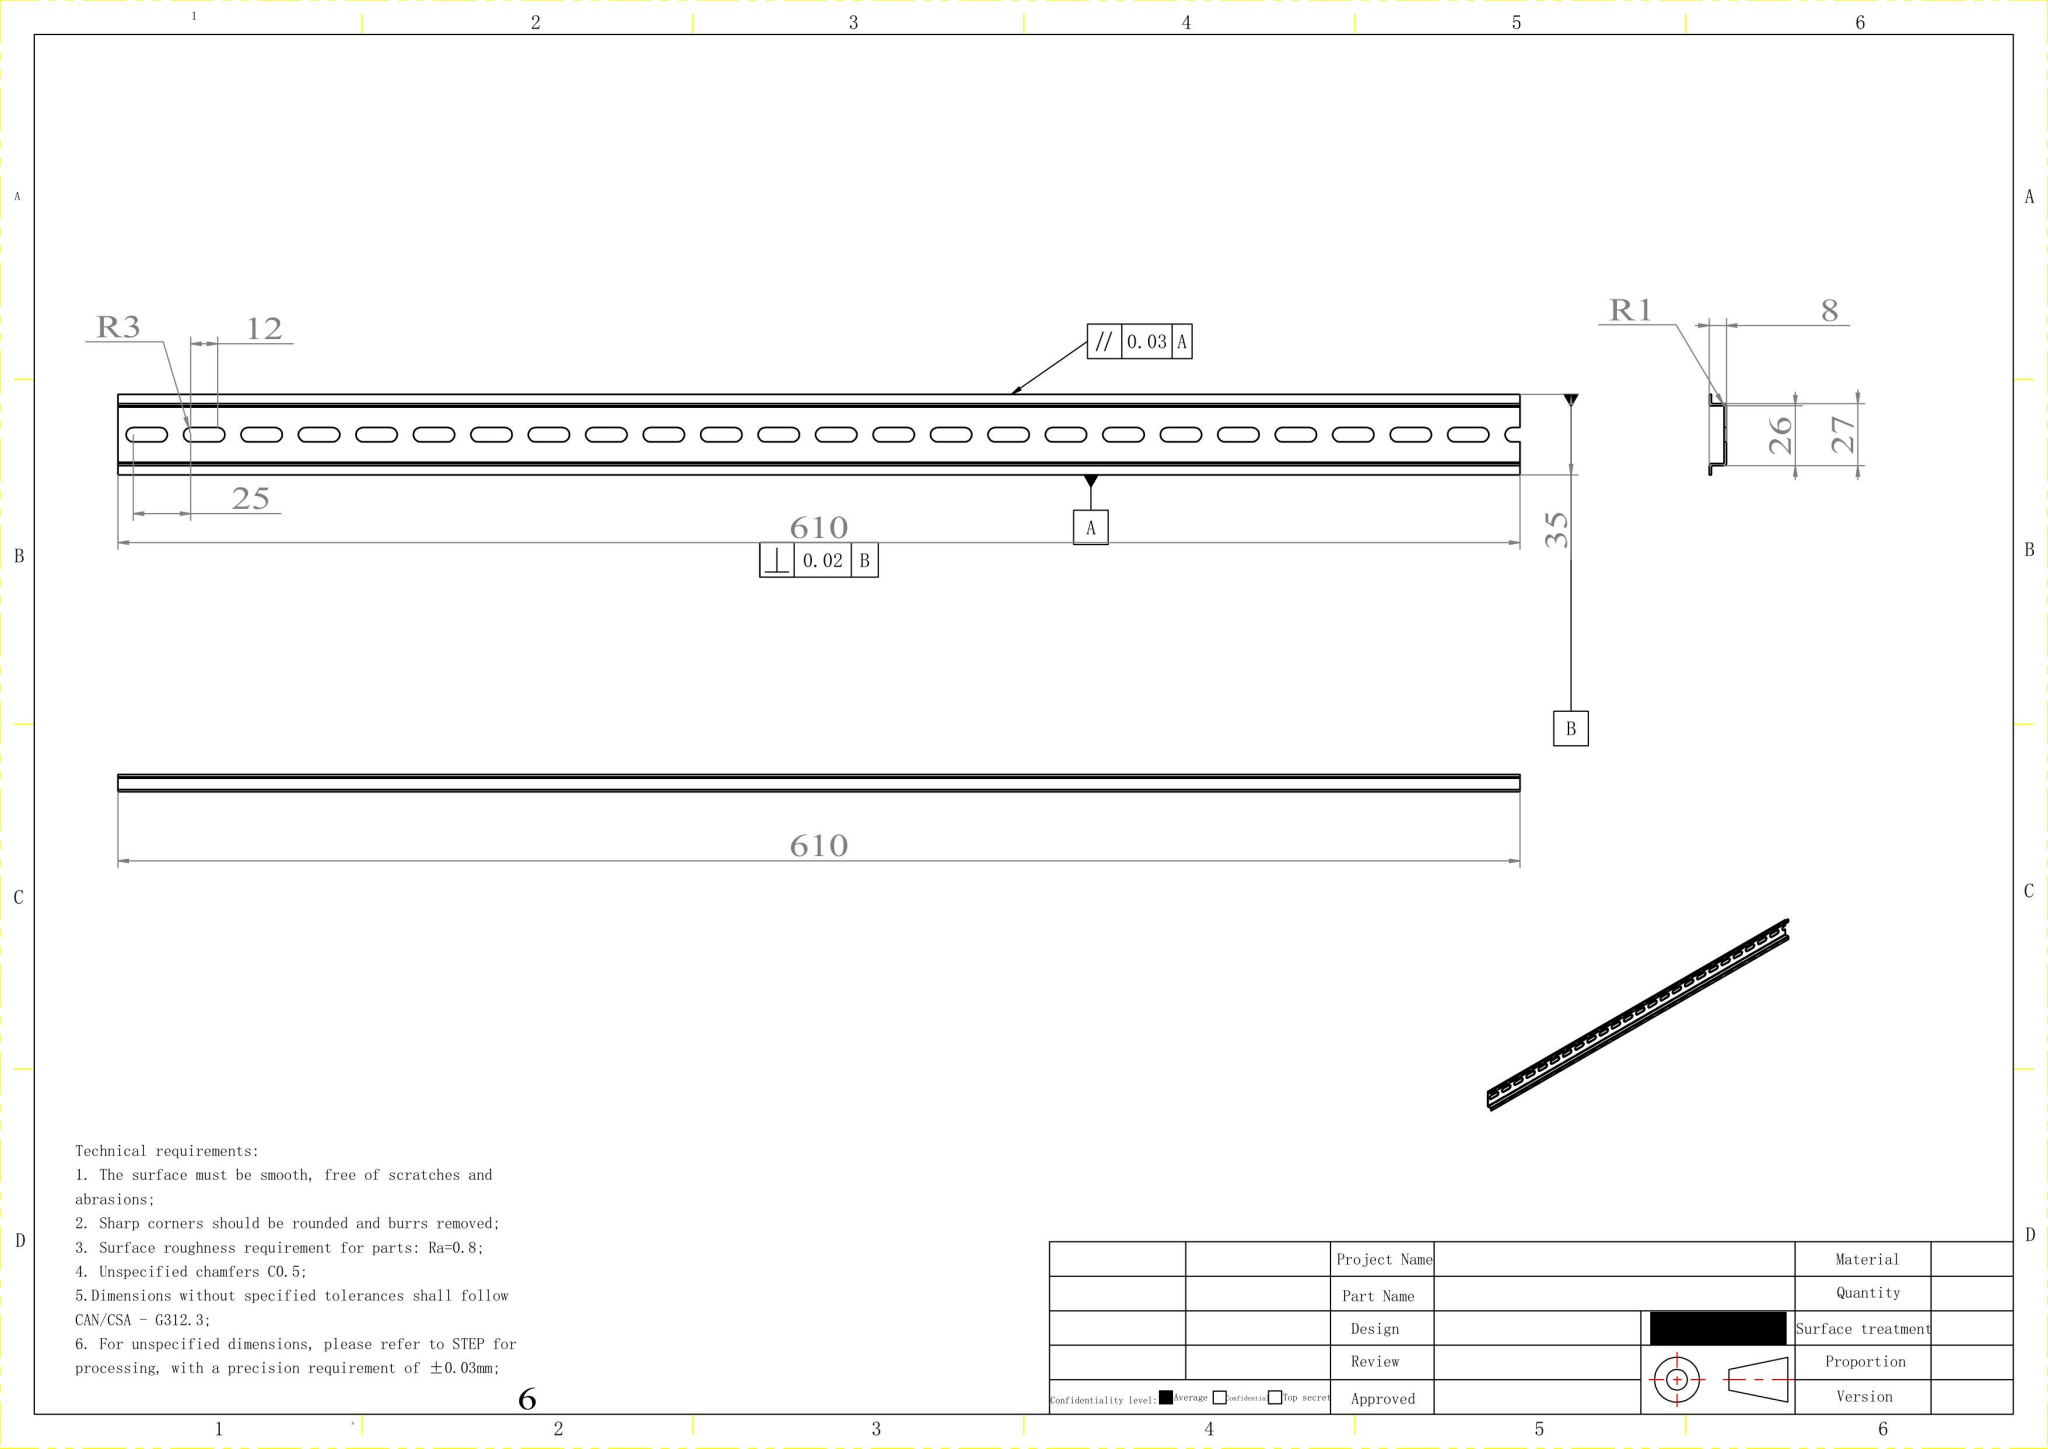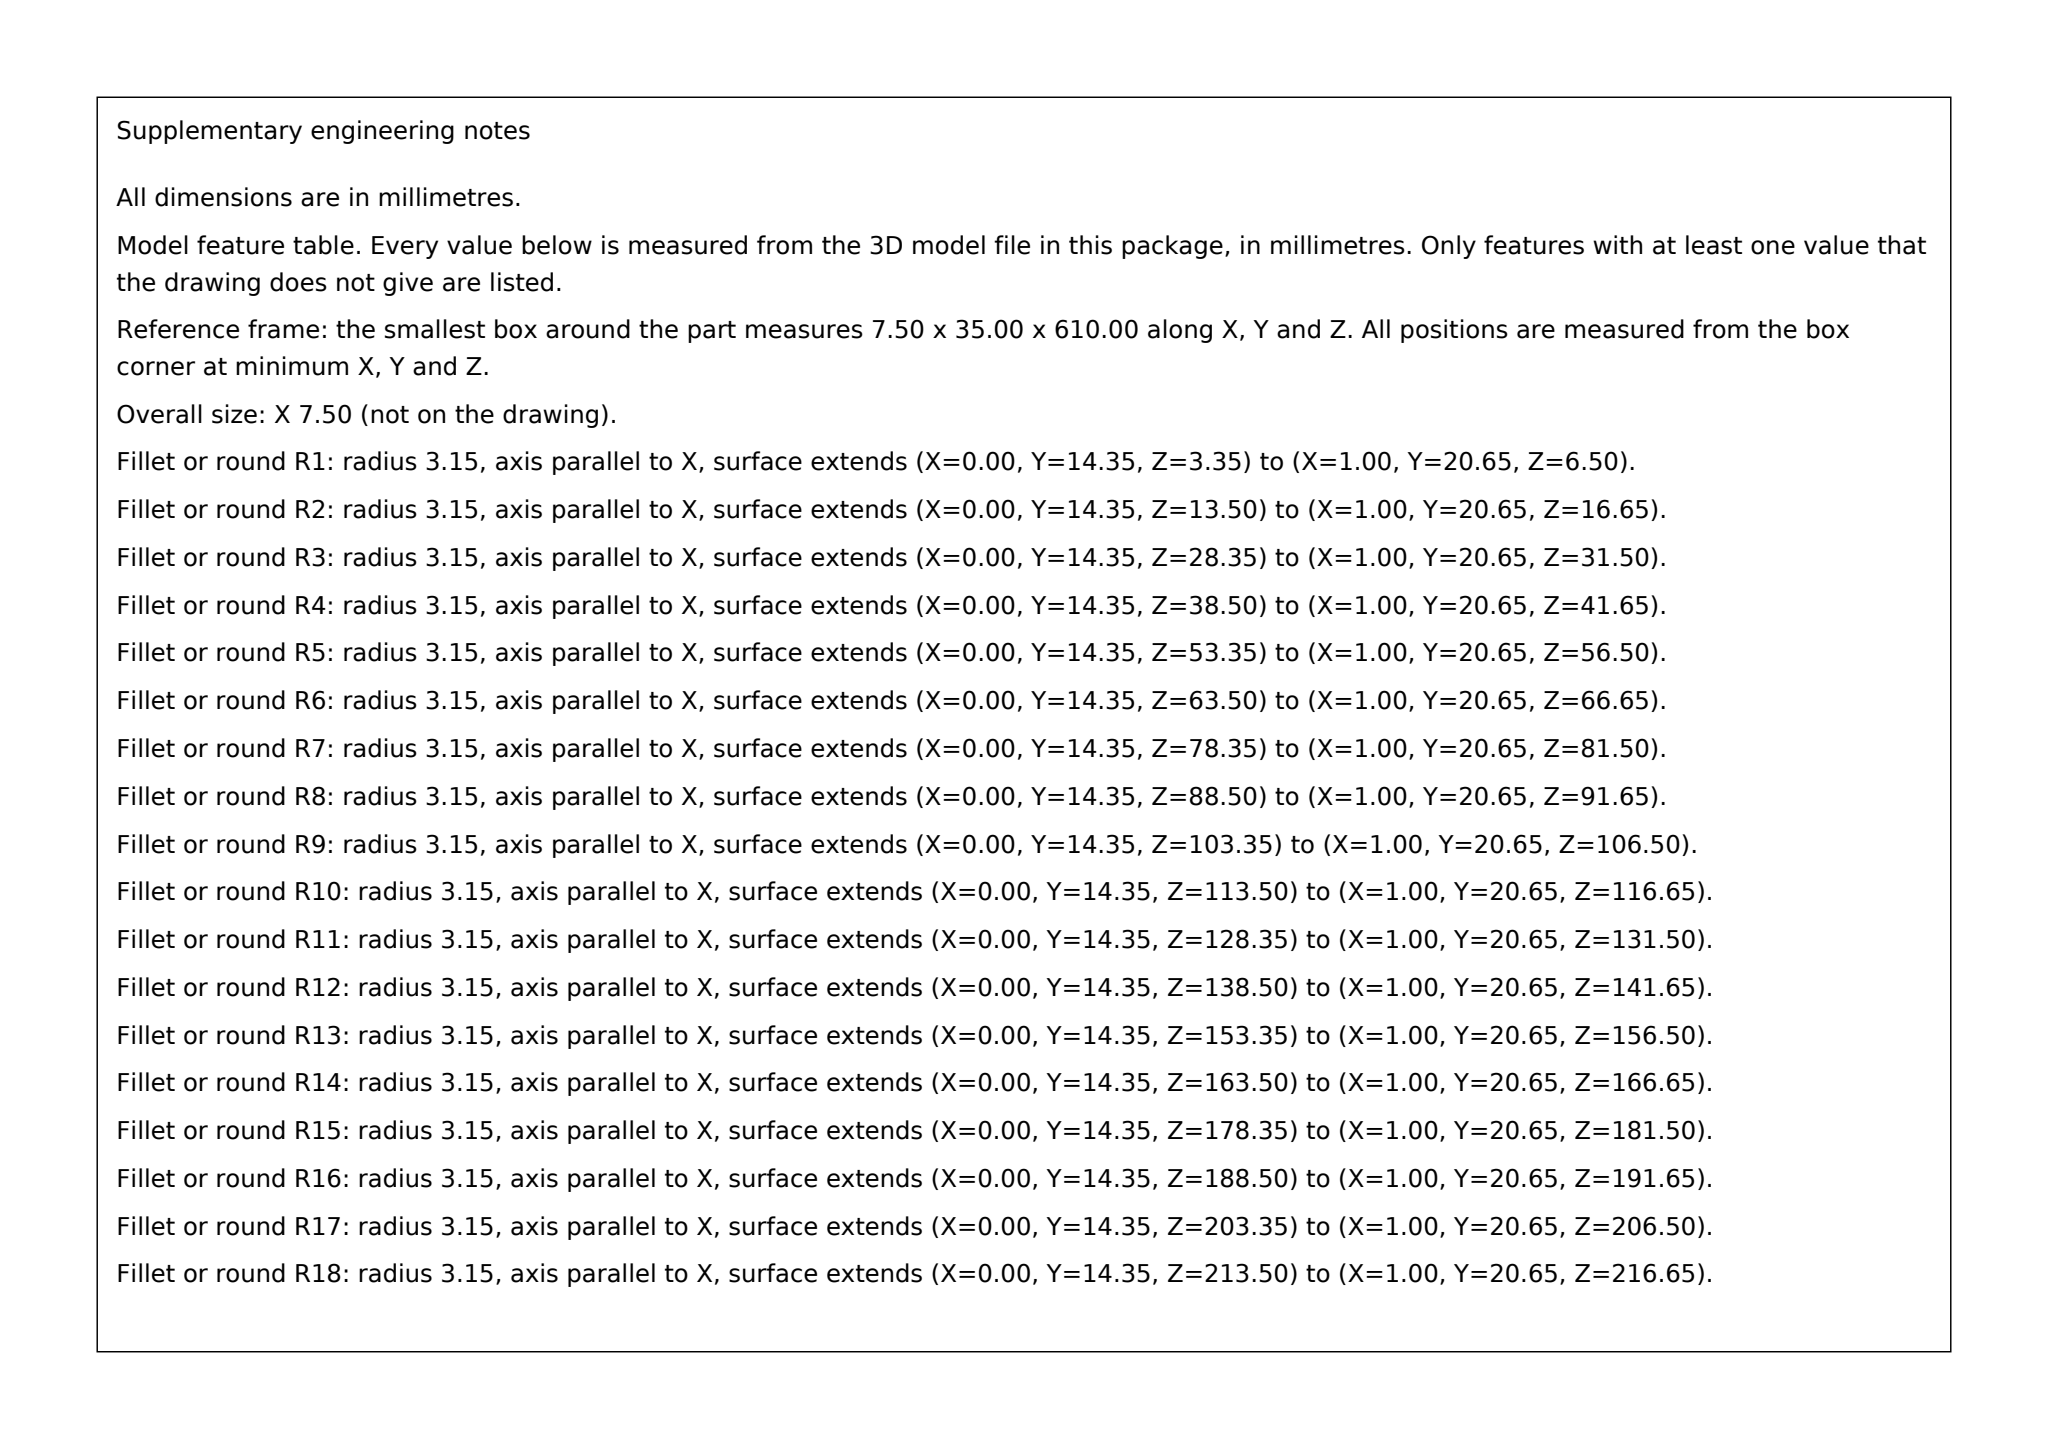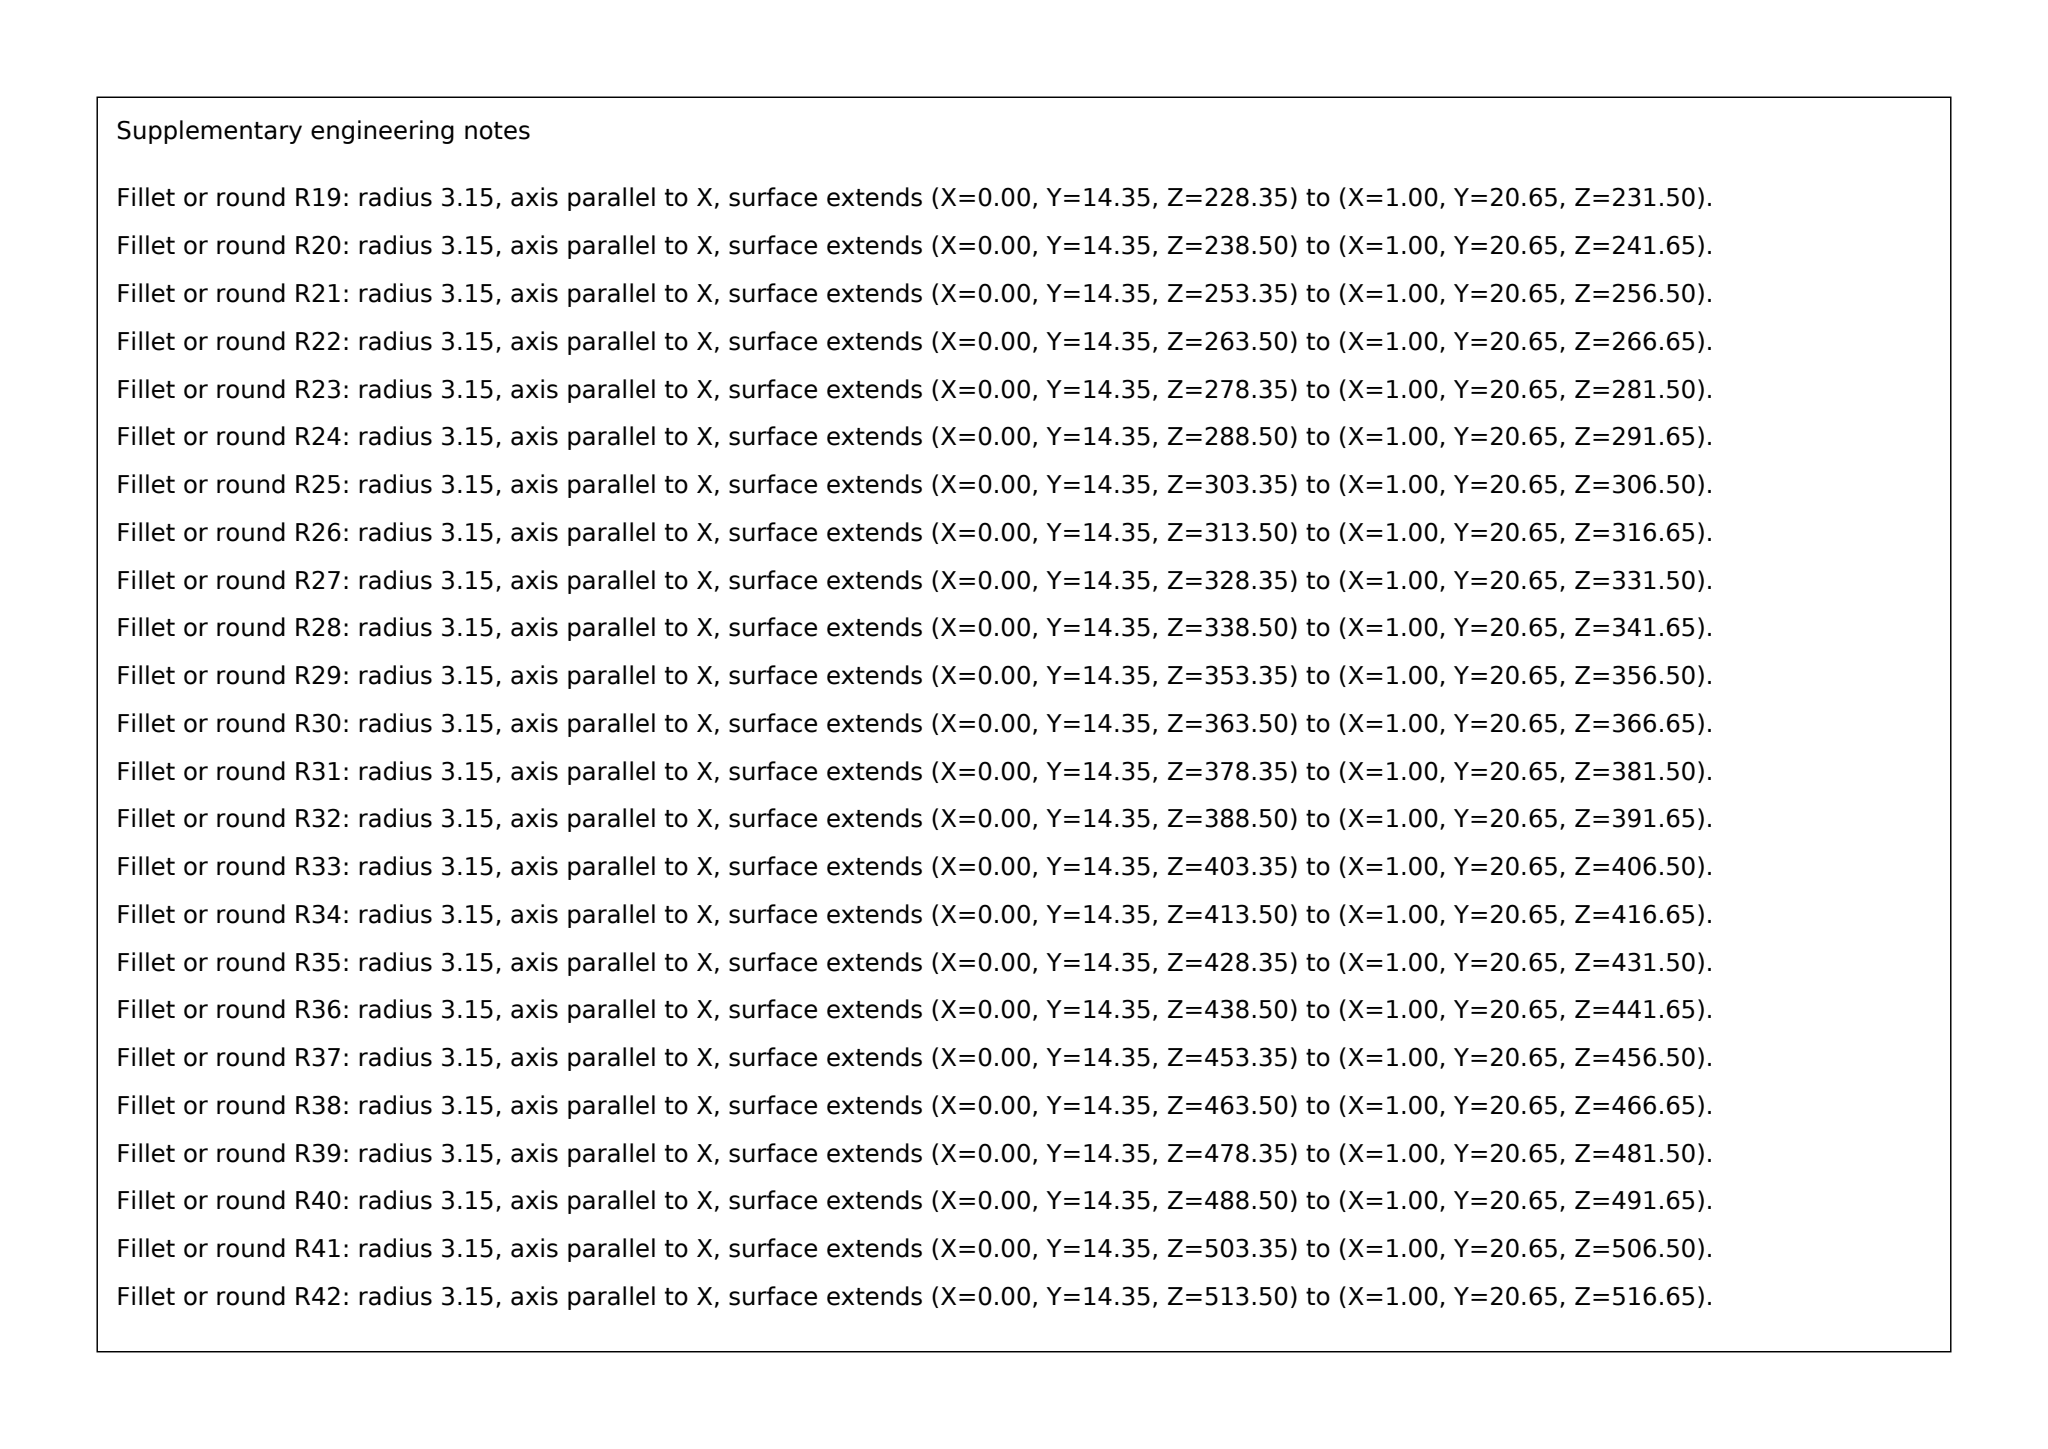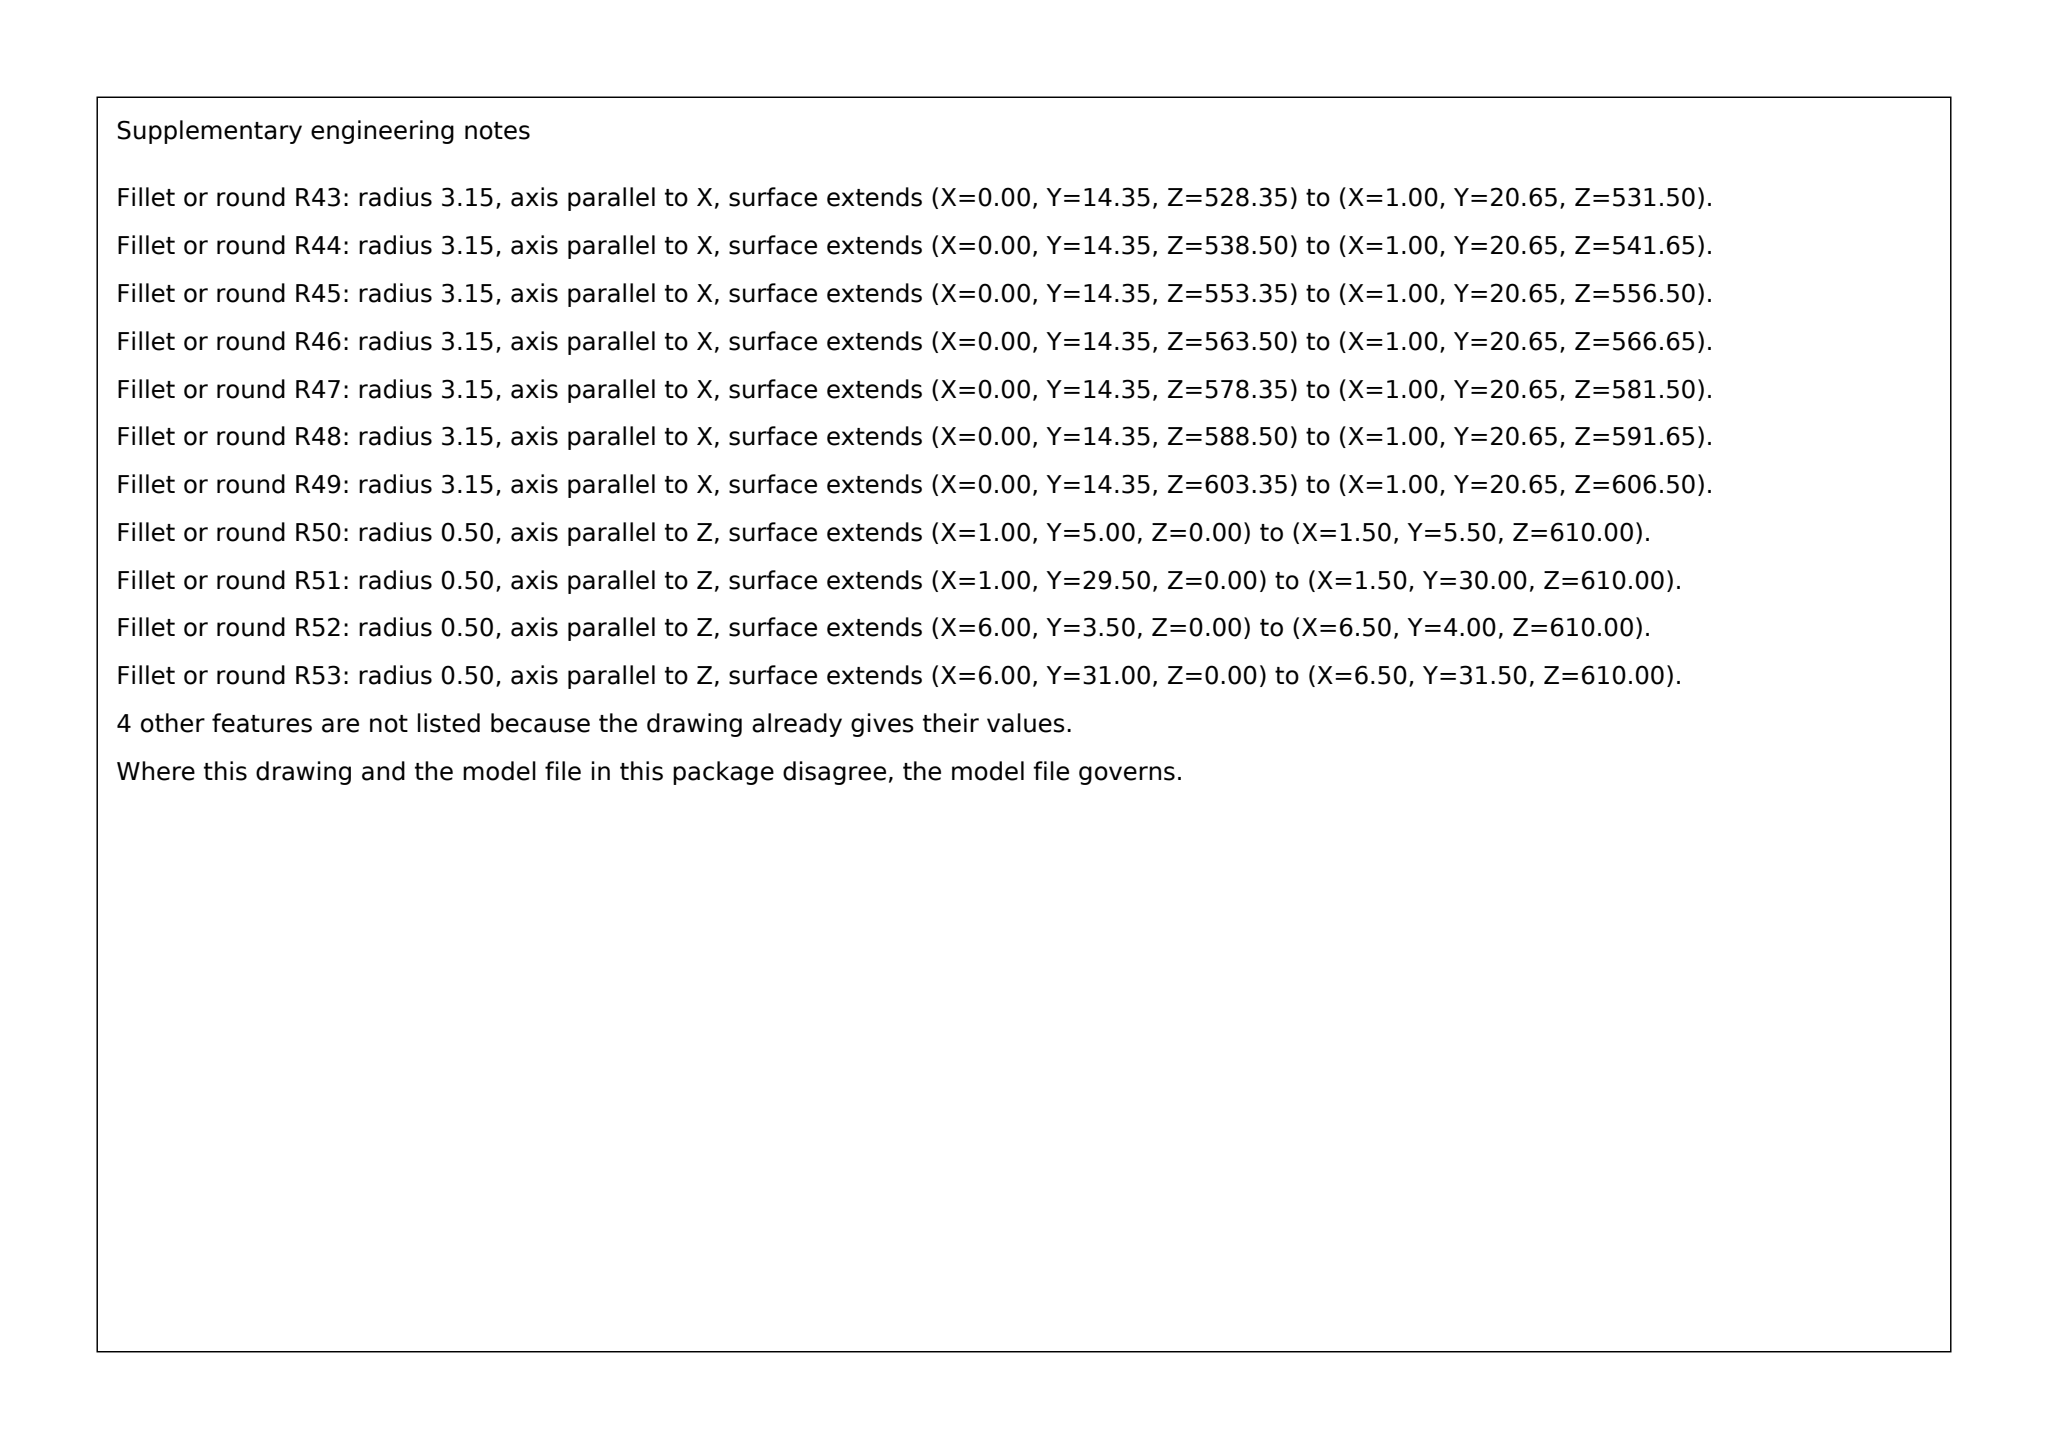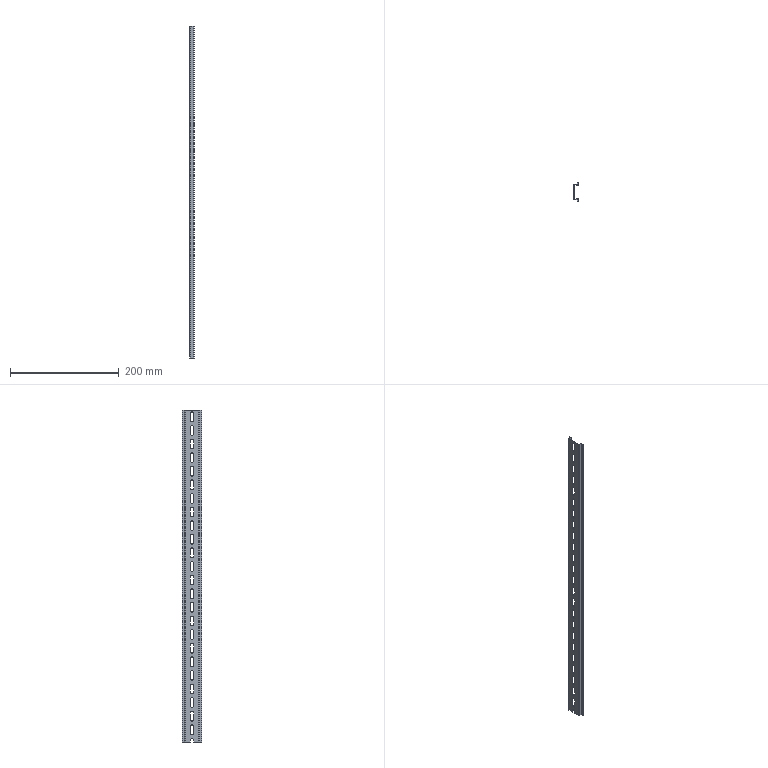Part | SolidWorks | mm | 1 solid | 122 faces | box 7.5 x 35 x 610 mm | volume 26333 mm3 | plane 65 | cylinder 57 | commonest cylinder face diameters 6.3 x49 2 x4 1 x4